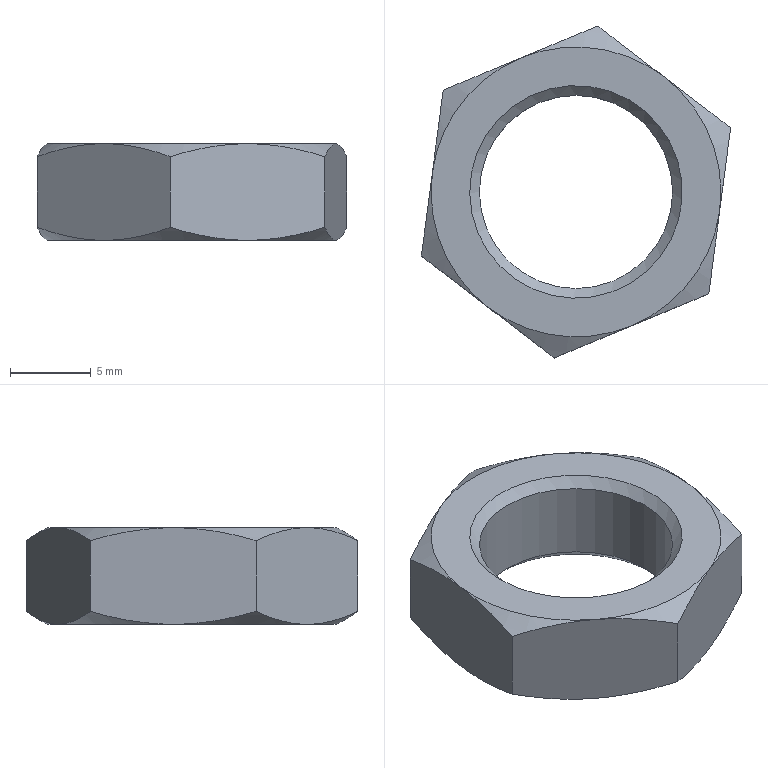Component | NX | NUT_M12 | 1 solid | 23 faces | volume 978 mm3 | cone 14 | plane 8 | cylinder 1 | commonest cylinder face diameters 12 x1